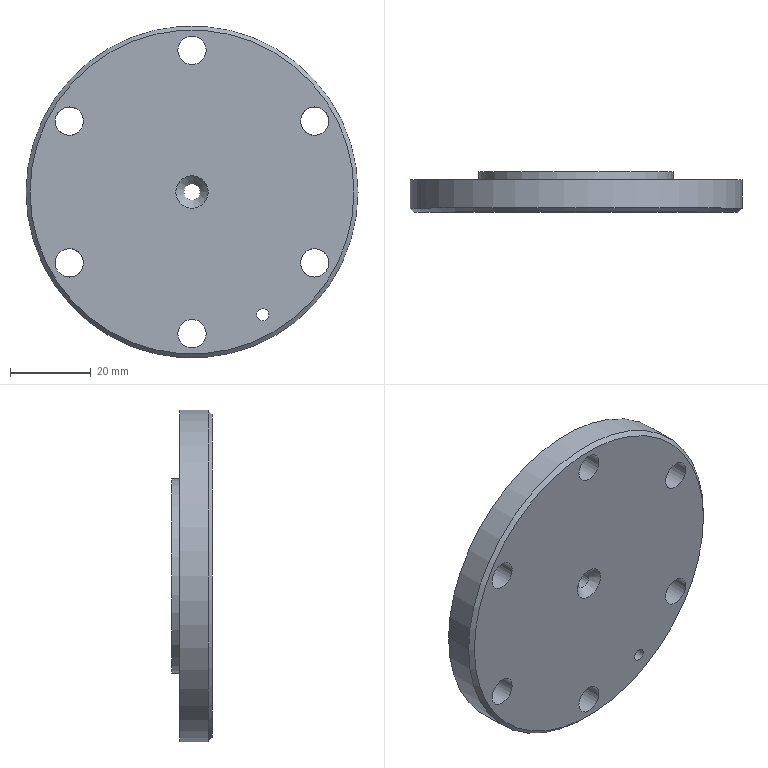Component | NX | PUMP_COVER | 1 solid | 15 faces | volume 43677 mm3 | cylinder 10 | plane 3 | cone 2 | commonest cylinder face diameters 7 x6 48 x1 82 x1 3 x1 4 x1